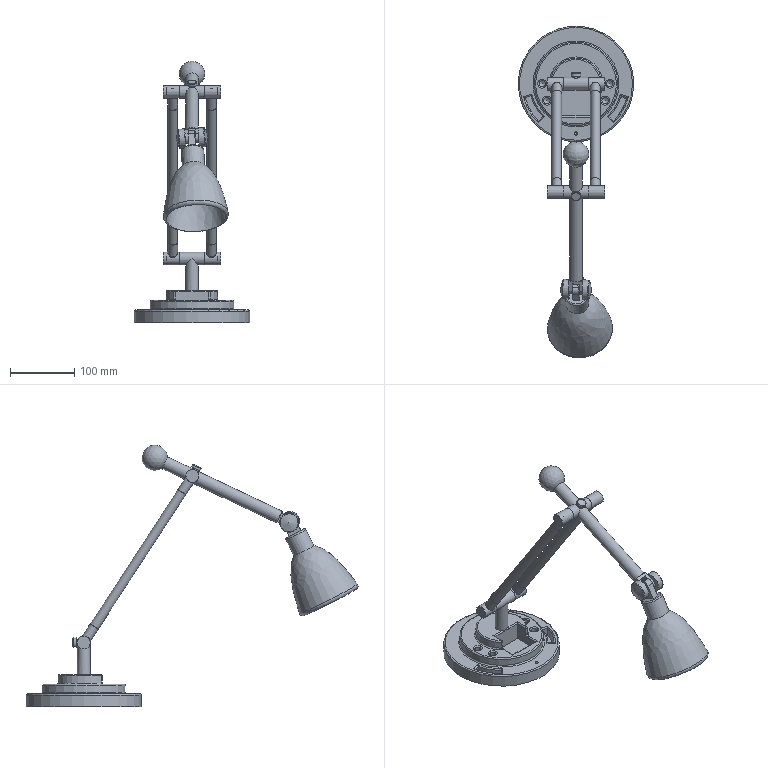Assembly | NX | mm | 17 component files | 19 solids | 237 faces | box 180 x 517.35 x 407.6 mm | volume 1126615 mm3 | cylinder 94 | plane 88 | torus 21 | cone 14 | spline 13 | other 4 | sphere 3 | commonest cylinder face diameters 10 x16 4 x15 15 x12 20 x10 16 x8 12 x8 6 x8 8.5 x4
Bill of materials:
unnamed part 1 | 1 |  | Stepped circular base with three coaxial tiers. A vertical post rises from the top tier and ends in a short horizontal hollow tube, giving a T shape. The base has a rectangular pocket, several holes and arc-shaped slots.
unnamed part 2 | 1 |  | Long straight rod with a sphere at one end and a short cross tube set crosswise near the sphere end. The far end of the rod is hollow.
unnamed part 3 | 2 |  | Short cylindrical disc with a central hole on one flat face. The opposite side tapers into a cone.
unnamed part 4 | 4 |  | Solid T-shaped body: a larger cylinder with a smaller cylinder sticking out sideways from its curved surface.
unnamed part 5 | 1 |  | Plain solid straight cylindrical rod with flat ends.
unnamed part 6 | 1 |  | Fork-shaped body: a rectangular block with two parallel lugs with rounded ends, each with an aligned cross hole, and a slot between them. A cylindrical shank extends from the opposite side of the block.
unnamed part 7 | 1 |  | Hollow dome- or bell-shaped thin shell, open at the wide end. A cylindrical neck at the narrow end carries a flat tab with a small hole.
unnamed part 8 | 2 |  | Slender stepped pin: a long cylindrical body that steps down twice to smaller-diameter ends at both ends.
unnamed part 9 | 2 |  | Solid cylindrical pin with chamfered ends and two radial cross holes, one near each end.
unnamed part 10 | 2 |  | Solid stepped cylinder: a larger-diameter head with a rounded outer edge and a smaller coaxial cylindrical shank.
Mates:
1. fix | Base_Plate 1 component
2. touch align | Key 2 face | Base_Plate 1 face
3. center | Key 2 face | Key 2 face | Base_Plate 1 face | Base_Plate 1 face
4. touch align | Cap 4 face | Key 2 face
5. touch align | Key 2 face | Cap 4 face
6. touch align | Cap 4 face | Bottom_Rod 2 face
7. touch align | Bottom_Rod 2 face | Cap 4 face
8. touch align | Key 2 face | Cap 3 face
9. touch align | Cap 3 face | Key 2 face
10. touch align | Bottom_Rod 1 face | Cap 3 face
11. touch align | Bottom_Rod 1 edge | Cap 3 edge
12. touch align | Key 1 face | Handle_Rod 1 face
13. touch align | Cap 1 face | Key 1 face
14. touch align | Key 1 face | Cap 1 face
15. touch align | Key 1 face | Cap 1 face
16. touch align | Cap 2 face | Key 1 face
17. touch align | Cap 2 face | Key 1 face
18. touch align | Cap 2 face | Key 1 face
19. touch align | Cap 2 face | Bottom_Rod 2 face
20. touch align | Cap 2 face | Bottom_Rod 2 face
21. touch align | Joint 1 face | Handle_Rod 1 face
22. center | Key2 1 face | Key2 1 face | Reflector 1 face | Reflector 1 face
23. touch align | Key2 1 face | Reflector 1 face
24. touch align | Key2 1 face | Joint 1 face
25. center | Key2 1 face | Key2 1 face | Joint 1 face | Joint 1 face
26. touch align | Cap2 2 | Key2 1 face
27. touch align | Cap2 2 face | Key2 1 face
28. touch align | Key2 1 face | Cap2 1
29. touch align | Key2 1 face | Cap2 1 face
30. fit | Bottom_Rod 2 face | Cap 4 face
31. touch align | Bolt 2 face | Handle_Rod 1 face
32. touch align | Bolt 2 face | Key 1 face
33. touch align | Bolt 1 face | Key 2 face
34. touch align | Bolt 1 face | Base_Plate 1 face
35. align lock | Bottom_Rod 1 face | Cap 1 face
36. align lock | Bottom_Rod 2 face | Cap 2 face
37. touch align | Joint 1 face | Handle_Rod 1
38. center | Handle_Rod 1 face | Handle_Rod 1 face | Key 1 face | Key 1 face